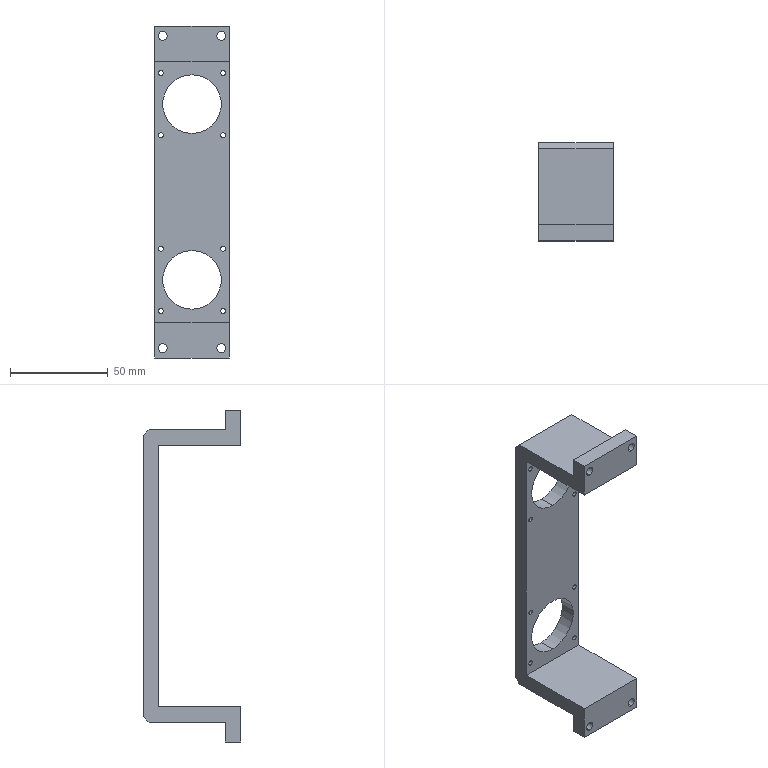Part | SolidWorks | mm | 1 solid | 44 faces | box 38 x 50 x 170 mm | volume 64741 mm3 | cylinder 28 | plane 16 | commonest cylinder face diameters 2.5 x16 4.5 x8 30 x4
Drawing notes:
4-Ø4.50 THRU ALL (8.00 THK FEET), NOT DP 20.00 | from the solid: 4x Ø4.5 holes, axis y, from y=0.0 to y=8.0 (full foot thk; y=0 and y=8 faces)
build123d program:
from build123d import *

# Parameters (mm, degrees)
BOSS_EXTRUDE1_DEPTH      = 19
SKETCH2_W                = 10
SKETCH2_H                = 8
BOSS_EXTRUDE2_DEPTH      = 38
CHAMFER1_SIZE            = 3
M4_CLEARANCE_HOLE1_D     = 4.5
M4_CLEARANCE_HOLE1_DEPTH = 20
M4_CLEARANCE_HOLE1_TIP   = 1.352
SKETCH6_R                = 15
CUT_EXTRUDE1_DEPTH       = 101.429
M3_TAPPED_HOLE1_D        = 2.5


with BuildPart() as part:
    # Sketch1 → Boss-Extrude1 (new, symmetric)
    with BuildSketch(Plane(origin=(0, 0, 0), x_dir=(0, 0, -1), z_dir=(1, 0, 0))):
        Polygon((-75, 25), (75, 25), (75, -25), (67, -25), (67, 17), (-67, 17), (-67, -25), (-75, -25), align=None)
    extrude(amount=BOSS_EXTRUDE1_DEPTH, both=True)

    # Sketch2 → Boss-Extrude2 (add)
    with BuildSketch(Plane(origin=(19, 0, 0), x_dir=(0, 0, -1), z_dir=(1, 0, 0))):
        with Locations((-80, -21)):
            Rectangle(SKETCH2_W, SKETCH2_H)
        with Locations((80, -21)):
            Rectangle(SKETCH2_W, SKETCH2_H)
    extrude(amount=-BOSS_EXTRUDE2_DEPTH)

    # Chamfer1
    chamfer1_edges = [part.edges().sort_by_distance(p)[0] for p in [
        (0, 25, -75),
        (0, 25, 75),
    ]]
    chamfer(chamfer1_edges, length=CHAMFER1_SIZE)

    # M4 Clearance Hole1
    with Locations(Plane(origin=(0, -17, 0), x_dir=(1, 0, 0), z_dir=(0, 1, 0))):
        with Locations((-15, 80), (15, 80), (-15, -80), (15, -80)):
            Hole(M4_CLEARANCE_HOLE1_D / 2, depth=M4_CLEARANCE_HOLE1_DEPTH)
            with Locations((0, 0, -(M4_CLEARANCE_HOLE1_DEPTH + M4_CLEARANCE_HOLE1_TIP / 2))):  # 118° drill point
                Cone(0, M4_CLEARANCE_HOLE1_D / 2, M4_CLEARANCE_HOLE1_TIP, mode=Mode.SUBTRACT)

    # Sketch6 → Cut-Extrude1 (cut, through all)
    with BuildSketch(Plane(origin=(0, 25, 0), x_dir=(1, 0, 0), z_dir=(0, 1, 0))):
        with Locations(Location((0, 45, 0), (0, 0, 270))):
            Circle(SKETCH6_R)
        with Locations(Location((0, -45, 0), (0, 0, 270))):
            Circle(SKETCH6_R)
    extrude(amount=-CUT_EXTRUDE1_DEPTH, mode=Mode.SUBTRACT)

    # M3 Tapped Hole1 (through all)
    with Locations(Plane(origin=(0, 25, 0), x_dir=(1, 0, 0), z_dir=(0, 1, 0))):
        with Locations((-15.91, 60.91), (15.91, 60.91), (15.91, 29.09), (-15.91, 29.09), (-15.91, -29.09), (-15.91, -60.91), (15.91, -60.91), (15.91, -29.09)):
            Hole(M3_TAPPED_HOLE1_D / 2)


solid = part.part